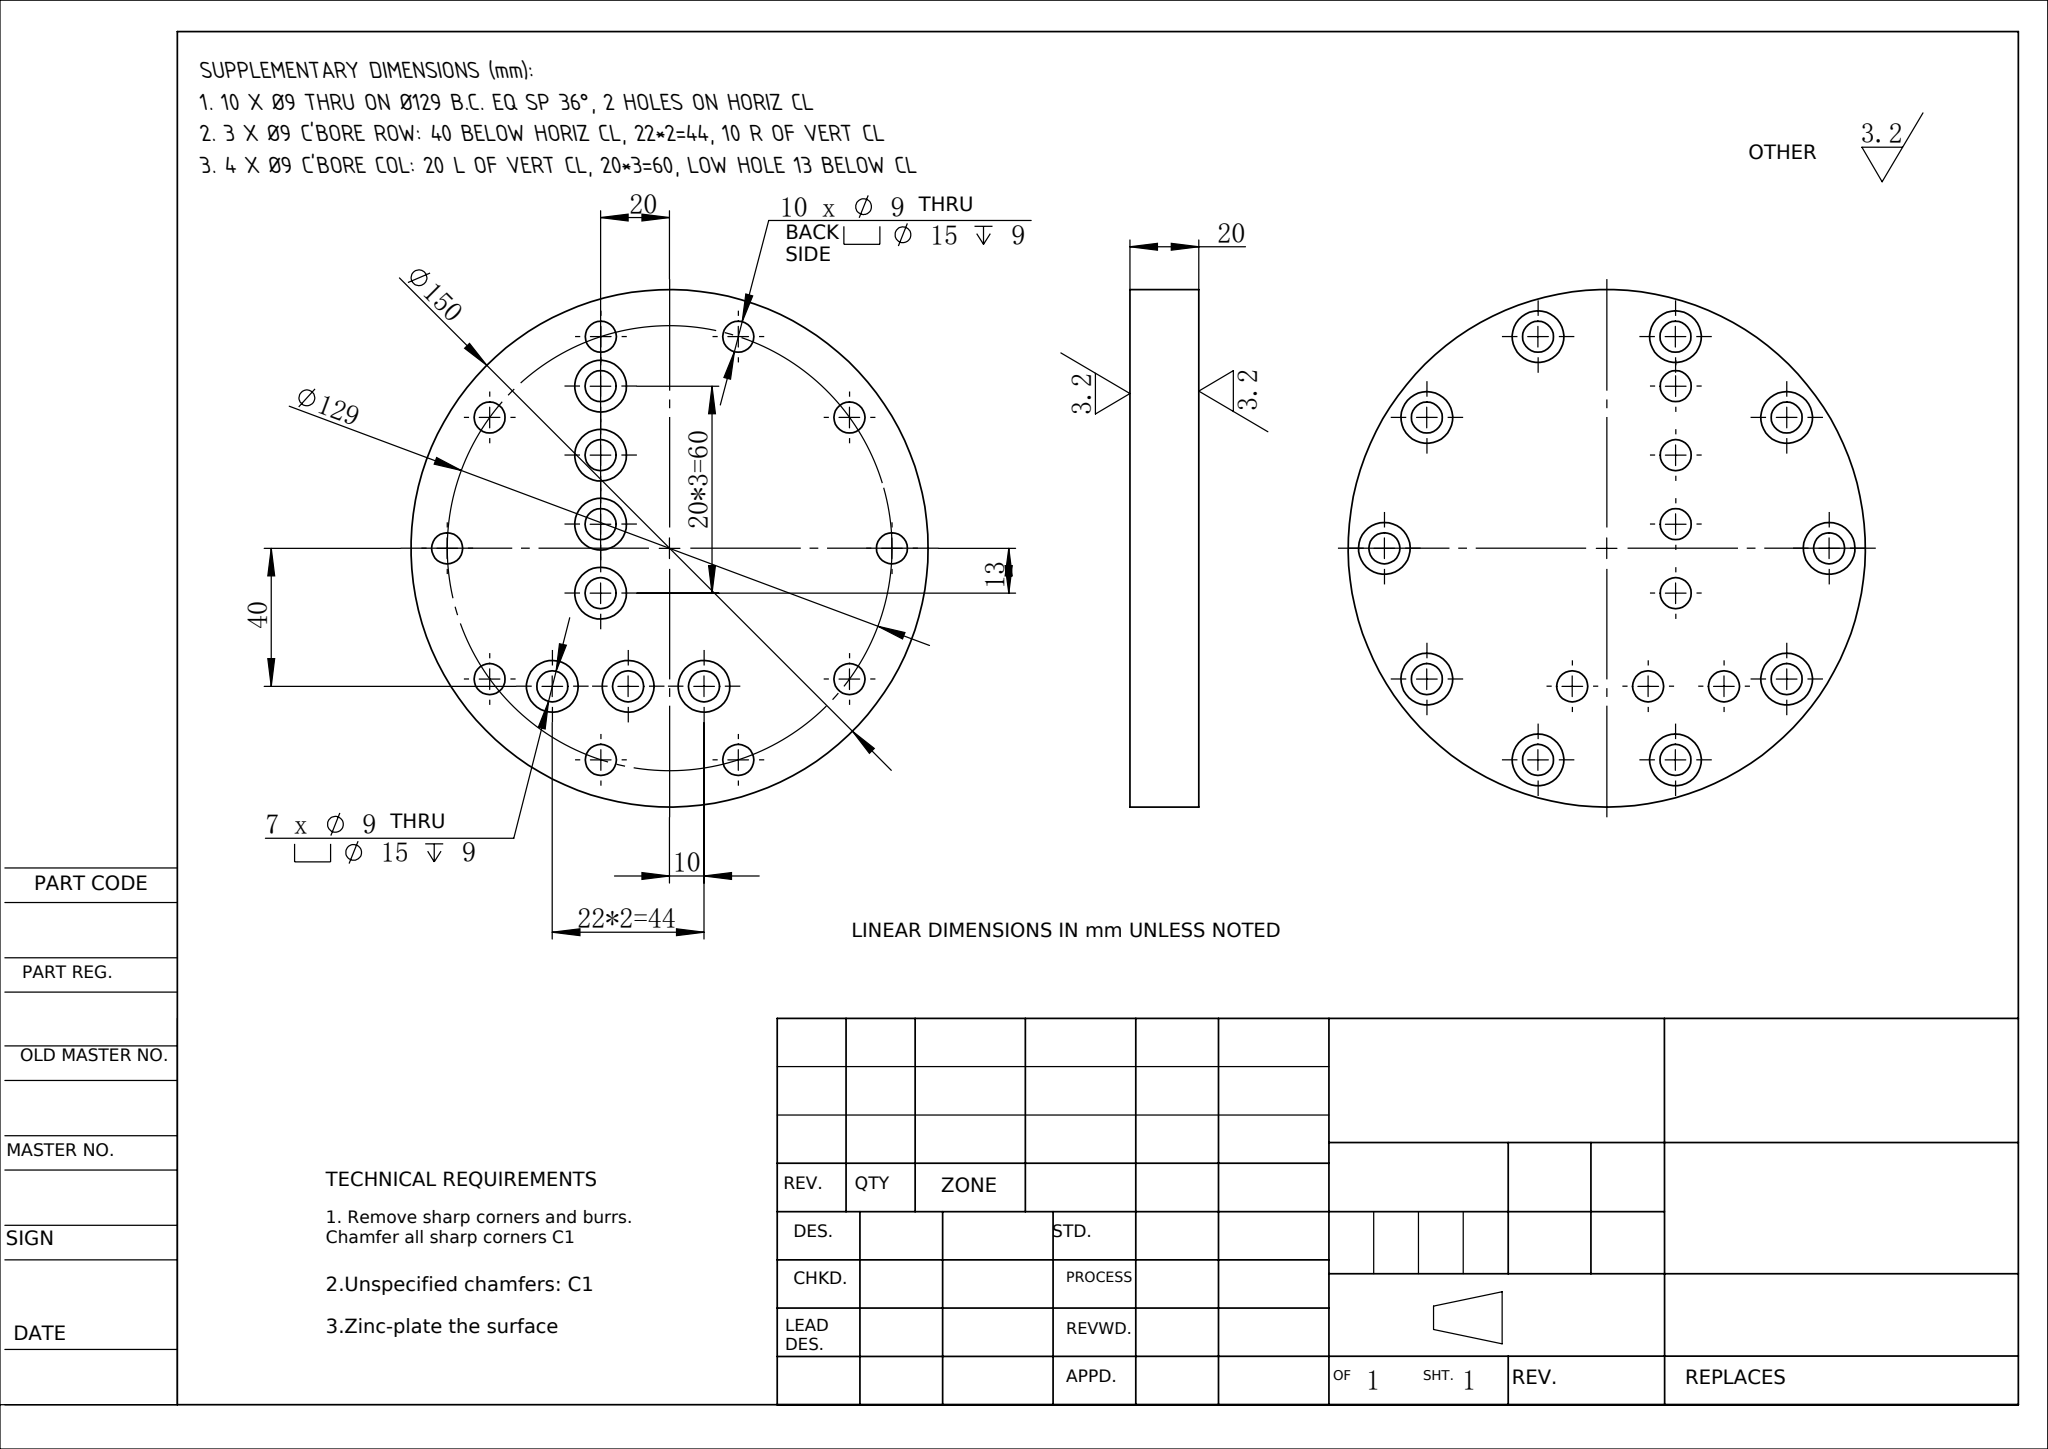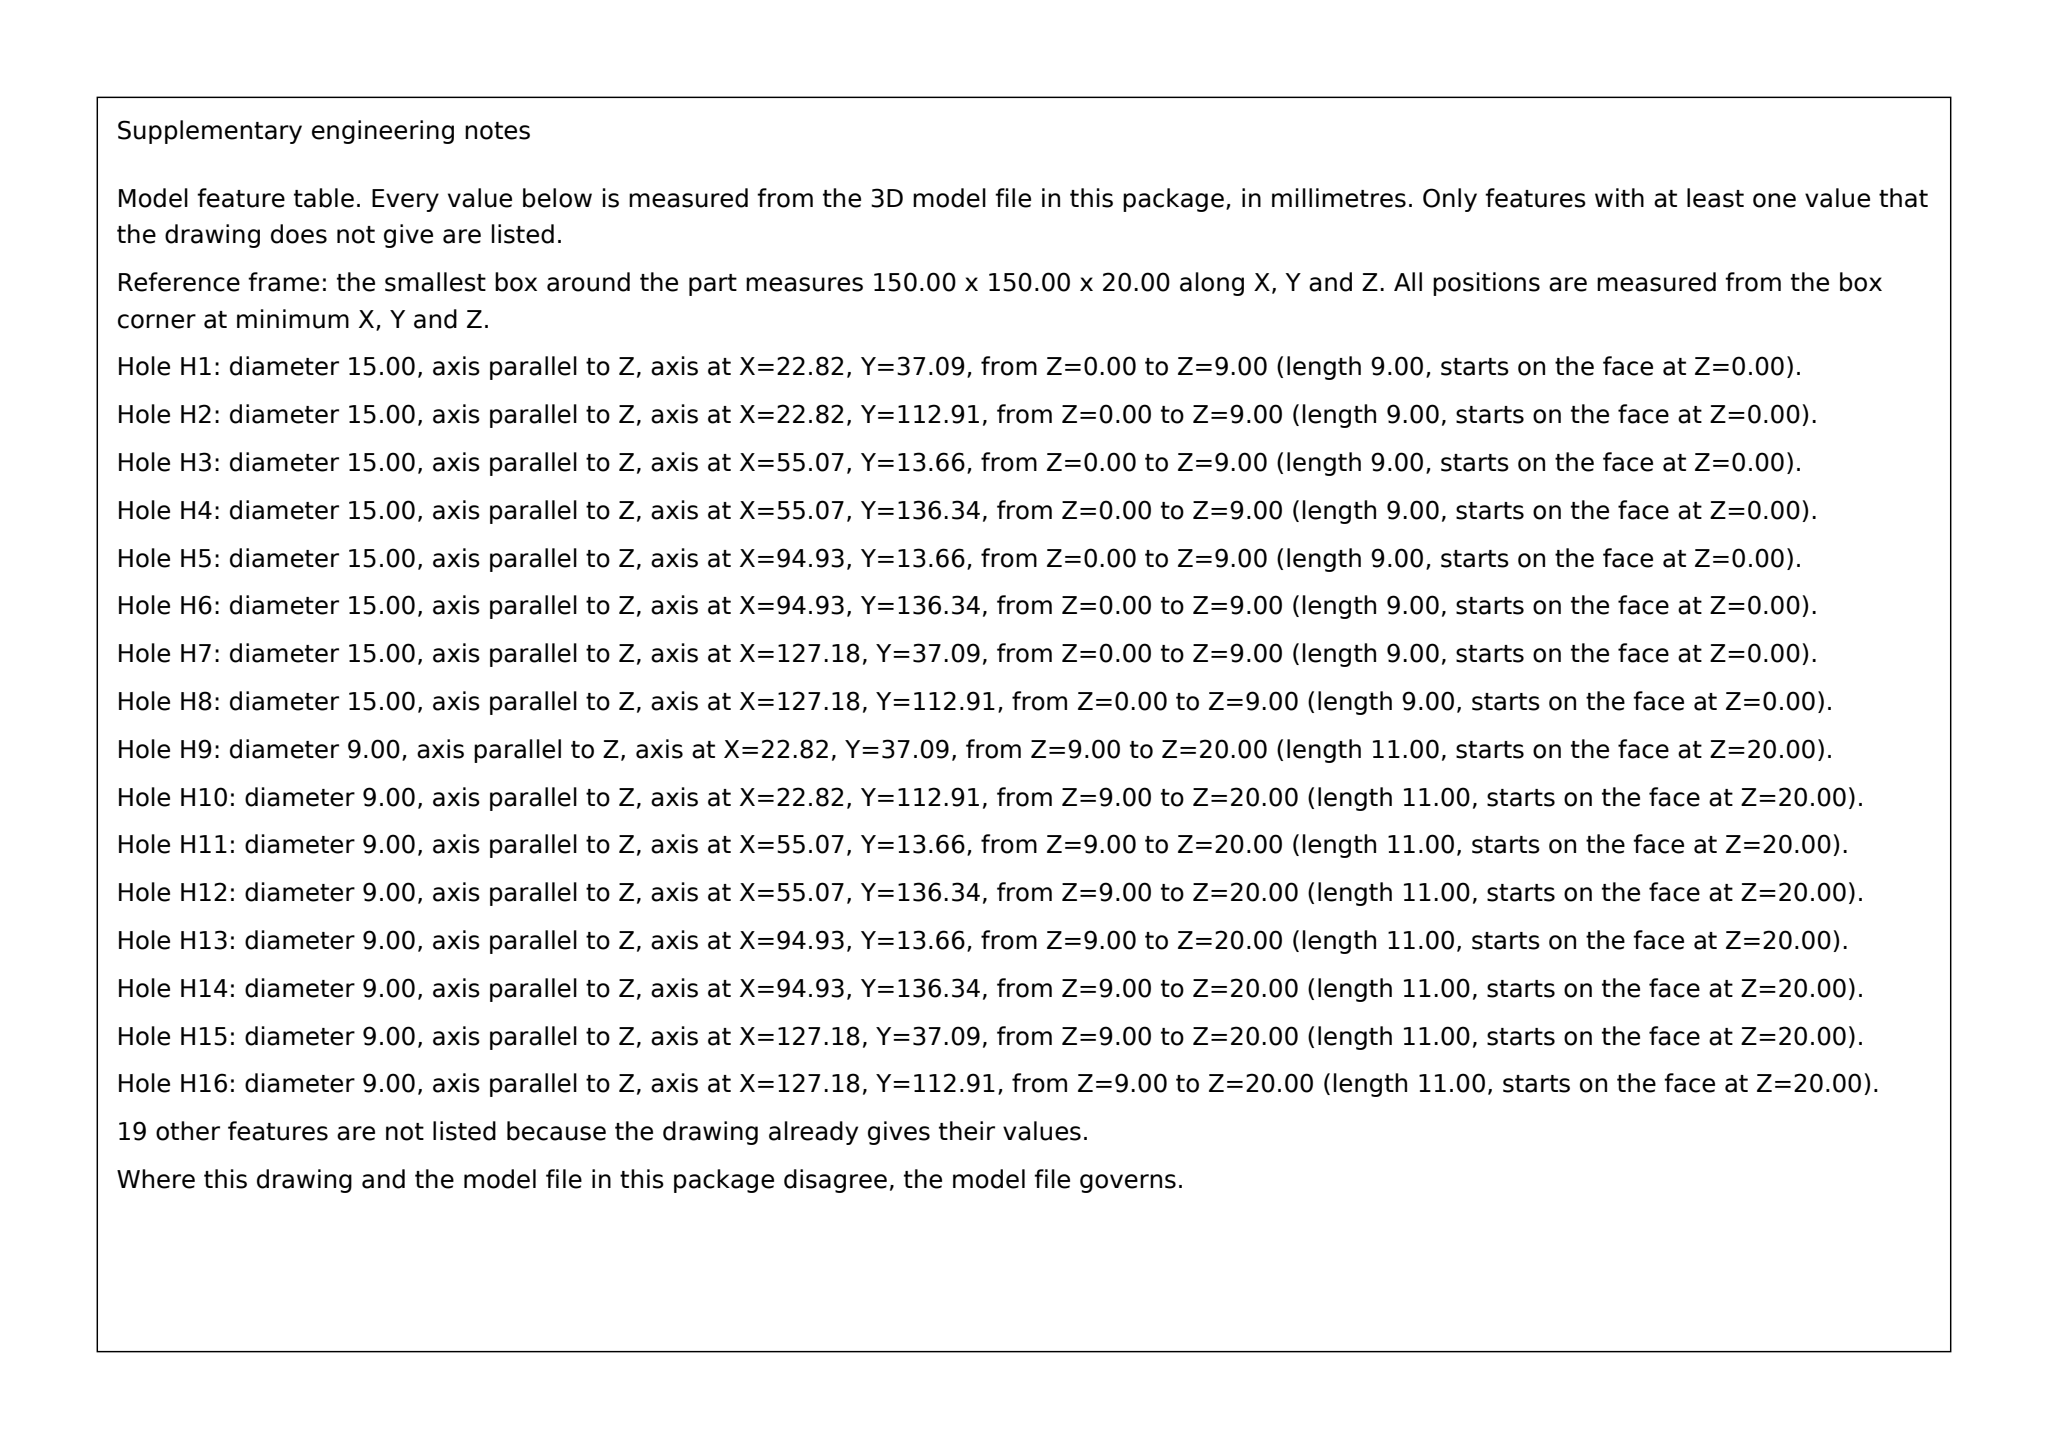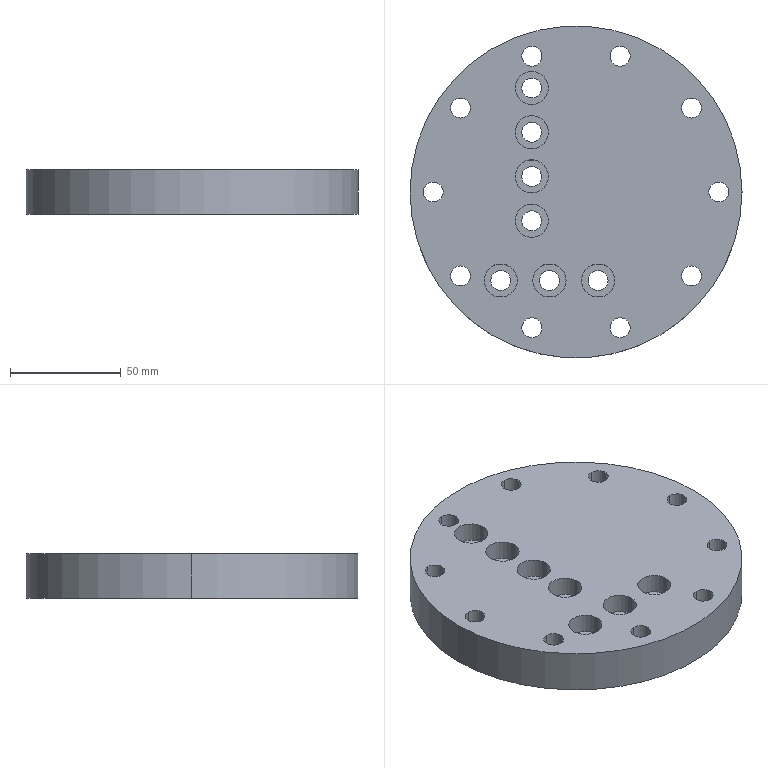Part | SolidWorks | mm | 1 solid | 89 faces | box 150 x 150 x 20 mm | volume 314495 mm3 | cylinder 70 | plane 19 | commonest cylinder face diameters 15 x34 9 x34 150 x2